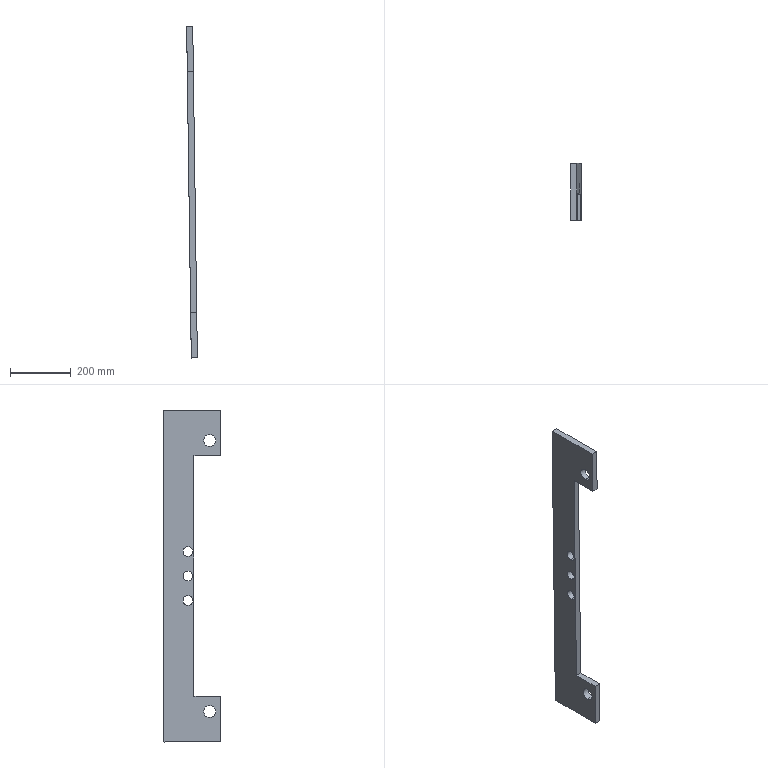Component | SolidWorks | DA-0220-Part3-1 | 1 solid | 22 faces | box 35.28 x 187.01 x 1090.17 mm | volume 2603445 mm3 | cylinder 12 | plane 10 | commonest cylinder face diameters 32 x6 40 x4 4 x2
build123d program:
from build123d import *

# Parameters (mm, degrees)
SKETCH1_W             = 1090
SKETCH1_H             = 100
BOSS_EXTRUDE1_DEPTH   = 20
FILLET1_R             = 2
SKETCH2_R             = 16
CUT_EXTRUDE2_DEPTH    = 548.654
SKETCH3_W             = 150
SKETCH3_H             = 87
BOSS_EXTRUDE1_2_DEPTH = 20
SKETCH4_R             = 20
CUT_EXTRUDE5_DEPTH    = 563.311


with BuildPart() as part:
    # Sketch1 → Boss-Extrude1 (new body)
    with BuildSketch(Plane.XY):
        Rectangle(SKETCH1_W, SKETCH1_H)
    extrude(amount=BOSS_EXTRUDE1_DEPTH)

    # Fillet1
    fillet1_edges = [part.edges().sort_by_distance(p)[0] for p in [
        (-545, 50, 10),
        (545, 50, 10),
    ]]
    fillet(fillet1_edges, radius=FILLET1_R)

    # Sketch2 → Cut-Extrude2 (cut, through all)
    with BuildSketch(Plane.XY.offset(20)):
        with Locations(Location((0, -30, 0), (0, 0, 180))):
            Circle(SKETCH2_R)
        with Locations((-80, -30)):
            Circle(SKETCH2_R)
        with Locations((80, -30)):
            Circle(SKETCH2_R)
    extrude(amount=-CUT_EXTRUDE2_DEPTH, mode=Mode.SUBTRACT)

    # Sketch3 → Boss-Extrude1_2 (add)
    with BuildSketch(Plane(origin=(0, 0, 0), x_dir=(-1, 0, 0), z_dir=(0, 0, -1))):
        with Locations((470, -93.5)):
            Rectangle(SKETCH3_W, SKETCH3_H)
        with Locations((-470, -93.5)):
            Rectangle(SKETCH3_W, SKETCH3_H)
    extrude(amount=-BOSS_EXTRUDE1_2_DEPTH)

    # Sketch4 → Cut-Extrude5 (cut, through all)
    with BuildSketch(Plane.XY.offset(20)):
        with Locations((-445, -102)):
            Circle(SKETCH4_R)
        with Locations((445, -102)):
            Circle(SKETCH4_R)
    extrude(amount=-CUT_EXTRUDE5_DEPTH, mode=Mode.SUBTRACT)


solid = part.part

# Placed as in the assembly
solid = solid.moved(Location((496.12, -63.852, 10.424), (178.341, -89.2, 178.341)))
STEP:
#1=CARTESIAN_POINT('',(18.98,-6.53,-16.331));
#2=VERTEX_POINT('',#1);
#3=CARTESIAN_POINT('',(19.002,-6.53,-17.906));
#4=VERTEX_POINT('',#3);
#5=CARTESIAN_POINT('',(18.991,-6.53,-17.119));
#6=DIRECTION('',(0.9999,0.000404,0.01395));
#7=DIRECTION('',(0.01395,0.00000282,-0.9999));
#8=AXIS2_PLACEMENT_3D('',#5,#6,#7);
#9=CIRCLE('',#8,0.7874);
#10=EDGE_CURVE('',#2,#4,#9,.T.);
#11=ORIENTED_EDGE('',*,*,#10,.F.);
#12=CARTESIAN_POINT('',(19.767,-6.53,-16.32));
#13=VERTEX_POINT('',#12);
#14=CARTESIAN_POINT('',(18.98,-6.53,-16.331));
#15=DIRECTION('',(0.9999,0.000404,0.01395));
#16=VECTOR('',#15,39.37);
#17=LINE('',#14,#16);
#18=EDGE_CURVE('',#2,#13,#17,.T.);
#19=ORIENTED_EDGE('',*,*,#18,.T.);
#20=CARTESIAN_POINT('',(19.789,-6.53,-17.895));
#21=VERTEX_POINT('',#20);
#22=CARTESIAN_POINT('',(19.778,-6.53,-17.108));
#23=DIRECTION('',(0.9999,0.000404,0.01395));
#24=DIRECTION('',(0.01395,0.00000282,-0.9999));
#25=AXIS2_PLACEMENT_3D('',#22,#23,#24);
#26=CIRCLE('',#25,0.7874);
#27=EDGE_CURVE('',#13,#21,#26,.T.);
#28=ORIENTED_EDGE('',*,*,#27,.T.);
#29=CARTESIAN_POINT('',(19.002,-6.53,-17.906));
#30=DIRECTION('',(0.9999,0.000404,0.01395));
#31=VECTOR('',#30,39.37);
#32=LINE('',#29,#31);
#33=EDGE_CURVE('',#4,#21,#32,.T.);
#34=ORIENTED_EDGE('',*,*,#33,.F.);
#35=EDGE_LOOP('',(#11,#19,#28,#34));
#36=FACE_OUTER_BOUND('',#35,.T.);
#37=CARTESIAN_POINT('',(18.991,-6.53,-17.119));
#38=DIRECTION('',(0.9999,0.000404,0.01395));
#39=DIRECTION('',(0.01395,0.00000282,-0.9999));
#40=AXIS2_PLACEMENT_3D('',#37,#38,#39);
#41=CYLINDRICAL_SURFACE('',#40,0.7874);
#42=ADVANCED_FACE('',(#36),#41,.F.);
#43=CARTESIAN_POINT('',(18.491,-6.53,18.705));
#44=VERTEX_POINT('',#43);
#45=CARTESIAN_POINT('',(18.513,-6.53,17.13));
#46=VERTEX_POINT('',#45);
#47=CARTESIAN_POINT('',(18.502,-6.53,17.917));
#48=DIRECTION('',(0.9999,0.000404,0.01395));
#49=DIRECTION('',(0.01395,0.00000282,-0.9999));
#50=AXIS2_PLACEMENT_3D('',#47,#48,#49);
#51=CIRCLE('',#50,0.7874);
#52=EDGE_CURVE('',#44,#46,#51,.T.);
#53=ORIENTED_EDGE('',*,*,#52,.F.);
#54=CARTESIAN_POINT('',(19.278,-6.53,18.716));
#55=VERTEX_POINT('',#54);
#56=CARTESIAN_POINT('',(18.491,-6.53,18.705));
#57=DIRECTION('',(0.9999,0.000404,0.01395));
#58=VECTOR('',#57,39.37);
#59=LINE('',#56,#58);
#60=EDGE_CURVE('',#44,#55,#59,.T.);
#61=ORIENTED_EDGE('',*,*,#60,.T.);
#62=CARTESIAN_POINT('',(19.3,-6.53,17.141));
#63=VERTEX_POINT('',#62);
#64=CARTESIAN_POINT('',(19.289,-6.53,17.928));
#65=DIRECTION('',(0.9999,0.000404,0.01395));
#66=DIRECTION('',(0.01395,0.00000282,-0.9999));
#67=AXIS2_PLACEMENT_3D('',#64,#65,#66);
#68=CIRCLE('',#67,0.7874);
#69=EDGE_CURVE('',#55,#63,#68,.T.);
#70=ORIENTED_EDGE('',*,*,#69,.T.);
#71=CARTESIAN_POINT('',(18.513,-6.53,17.13));
#72=DIRECTION('',(0.9999,0.000404,0.01395));
#73=VECTOR('',#72,39.37);
#74=LINE('',#71,#73);
#75=EDGE_CURVE('',#46,#63,#74,.T.);
#76=ORIENTED_EDGE('',*,*,#75,.F.);
#77=EDGE_LOOP('',(#53,#61,#70,#76));
#78=FACE_OUTER_BOUND('',#77,.T.);
#79=CARTESIAN_POINT('',(18.502,-6.53,17.917));
#80=DIRECTION('',(0.9999,0.000404,0.01395));
#81=DIRECTION('',(0.01395,0.00000282,-0.9999));
#82=AXIS2_PLACEMENT_3D('',#79,#80,#81);
#83=CYLINDRICAL_SURFACE('',#82,0.7874);
#84=ADVANCED_FACE('',(#78),#83,.F.);
#85=CARTESIAN_POINT('',(18.781,-3.695,-2.12));
#86=VERTEX_POINT('',#85);
#87=CARTESIAN_POINT('',(18.798,-3.695,-3.38));
#88=VERTEX_POINT('',#87);
#89=CARTESIAN_POINT('',(18.789,-3.695,-2.75));
#90=DIRECTION('',(0.9999,0.000404,0.01395));
#91=DIRECTION('',(0.01395,0.00000282,-0.9999));
#92=AXIS2_PLACEMENT_3D('',#89,#90,#91);
#93=CIRCLE('',#92,0.6299);
#94=EDGE_CURVE('',#86,#88,#93,.T.);
#95=ORIENTED_EDGE('',*,*,#94,.F.);
#96=CARTESIAN_POINT('',(19.568,-3.695,-2.109));
#97=VERTEX_POINT('',#96);
#98=CARTESIAN_POINT('',(18.781,-3.695,-2.12));
#99=DIRECTION('',(0.9999,0.000404,0.01395));
#100=VECTOR('',#99,39.37);
#101=LINE('',#98,#100);
#102=EDGE_CURVE('',#86,#97,#101,.T.);
#103=ORIENTED_EDGE('',*,*,#102,.T.);
#104=CARTESIAN_POINT('',(19.585,-3.695,-3.369));
#105=VERTEX_POINT('',#104);
#106=CARTESIAN_POINT('',(19.577,-3.695,-2.739));
#107=DIRECTION('',(0.9999,0.000404,0.01395));
#108=DIRECTION('',(0.01395,0.00000282,-0.9999));
#109=AXIS2_PLACEMENT_3D('',#106,#107,#108);
#110=CIRCLE('',#109,0.6299);
#111=EDGE_CURVE('',#97,#105,#110,.T.);
#112=ORIENTED_EDGE('',*,*,#111,.T.);
#113=CARTESIAN_POINT('',(18.798,-3.695,-3.38));
#114=DIRECTION('',(0.9999,0.000404,0.01395));
#115=VECTOR('',#114,39.37);
#116=LINE('',#113,#115);
#117=EDGE_CURVE('',#88,#105,#116,.T.);
#118=ORIENTED_EDGE('',*,*,#117,.F.);
#119=EDGE_LOOP('',(#95,#103,#112,#118));
#120=FACE_OUTER_BOUND('',#119,.T.);
#121=CARTESIAN_POINT('',(18.789,-3.695,-2.75));
#122=DIRECTION('',(0.9999,0.000404,0.01395));
#123=DIRECTION('',(0.01395,0.00000282,-0.9999));
#124=AXIS2_PLACEMENT_3D('',#121,#122,#123);
#125=CYLINDRICAL_SURFACE('',#124,0.6299);
#126=ADVANCED_FACE('',(#120),#125,.F.);
#127=CARTESIAN_POINT('',(18.693,-3.695,4.179));
#128=VERTEX_POINT('',#127);
#129=CARTESIAN_POINT('',(18.71,-3.695,2.919));
#130=VERTEX_POINT('',#129);
#131=CARTESIAN_POINT('',(18.701,-3.695,3.549));
#132=DIRECTION('',(0.9999,0.000404,0.01395));
#133=DIRECTION('',(0.01395,0.00000282,-0.9999));
#134=AXIS2_PLACEMENT_3D('',#131,#132,#133);
#135=CIRCLE('',#134,0.6299);
#136=EDGE_CURVE('',#128,#130,#135,.T.);
#137=ORIENTED_EDGE('',*,*,#136,.F.);
#138=CARTESIAN_POINT('',(19.48,-3.695,4.19));
#139=VERTEX_POINT('',#138);
#140=CARTESIAN_POINT('',(18.693,-3.695,4.179));
#141=DIRECTION('',(0.9999,0.000404,0.01395));
#142=VECTOR('',#141,39.37);
#143=LINE('',#140,#142);
#144=EDGE_CURVE('',#128,#139,#143,.T.);
#145=ORIENTED_EDGE('',*,*,#144,.T.);
#146=CARTESIAN_POINT('',(19.498,-3.695,2.93));
#147=VERTEX_POINT('',#146);
#148=CARTESIAN_POINT('',(19.489,-3.695,3.56));
#149=DIRECTION('',(0.9999,0.000404,0.01395));
#150=DIRECTION('',(0.01395,0.00000282,-0.9999));
#151=AXIS2_PLACEMENT_3D('',#148,#149,#150);
#152=CIRCLE('',#151,0.6299);
#153=EDGE_CURVE('',#139,#147,#152,.T.);
#154=ORIENTED_EDGE('',*,*,#153,.T.);
#155=CARTESIAN_POINT('',(18.71,-3.695,2.919));
#156=DIRECTION('',(0.9999,0.000404,0.01395));
#157=VECTOR('',#156,39.37);
#158=LINE('',#155,#157);
#159=EDGE_CURVE('',#130,#147,#158,.T.);
#160=ORIENTED_EDGE('',*,*,#159,.F.);
#161=EDGE_LOOP('',(#137,#145,#154,#160));
#162=FACE_OUTER_BOUND('',#161,.T.);
#163=CARTESIAN_POINT('',(18.701,-3.695,3.549));
#164=DIRECTION('',(0.9999,0.000404,0.01395));
#165=DIRECTION('',(0.01395,0.00000282,-0.9999));
#166=AXIS2_PLACEMENT_3D('',#163,#164,#165);
#167=CYLINDRICAL_SURFACE('',#166,0.6299);
#168=ADVANCED_FACE('',(#162),#167,.F.);
#169=CARTESIAN_POINT('',(18.737,-3.695,1.029));
#170=VERTEX_POINT('',#169);
#171=CARTESIAN_POINT('',(18.754,-3.695,-0.2304));
#172=VERTEX_POINT('',#171);
#173=CARTESIAN_POINT('',(18.745,-3.695,0.3994));
#174=DIRECTION('',(0.9999,0.000404,0.01395));
#175=DIRECTION('',(-0.01395,-0.00000282,0.9999));
#176=AXIS2_PLACEMENT_3D('',#173,#174,#175);
#177=CIRCLE('',#176,0.6299);
#178=EDGE_CURVE('',#170,#172,#177,.T.);
#179=ORIENTED_EDGE('',*,*,#178,.F.);
#180=CARTESIAN_POINT('',(19.524,-3.695,1.04));
#181=VERTEX_POINT('',#180);
#182=CARTESIAN_POINT('',(18.737,-3.695,1.029));
#183=DIRECTION('',(0.9999,0.000404,0.01395));
#184=VECTOR('',#183,39.37);
#185=LINE('',#182,#184);
#186=EDGE_CURVE('',#170,#181,#185,.T.);
#187=ORIENTED_EDGE('',*,*,#186,.T.);
#188=CARTESIAN_POINT('',(19.542,-3.695,-0.2194));
#189=VERTEX_POINT('',#188);
#190=CARTESIAN_POINT('',(19.533,-3.695,0.4104));
#191=DIRECTION('',(0.9999,0.000404,0.01395));
#192=DIRECTION('',(-0.01395,-0.00000282,0.9999));
#193=AXIS2_PLACEMENT_3D('',#190,#191,#192);
#194=CIRCLE('',#193,0.6299);
#195=EDGE_CURVE('',#181,#189,#194,.T.);
#196=ORIENTED_EDGE('',*,*,#195,.T.);
#197=CARTESIAN_POINT('',(18.754,-3.695,-0.2304));
#198=DIRECTION('',(0.9999,0.000404,0.01395));
#199=VECTOR('',#198,39.37);
#200=LINE('',#197,#199);
#201=EDGE_CURVE('',#172,#189,#200,.T.);
#202=ORIENTED_EDGE('',*,*,#201,.F.);
#203=EDGE_LOOP('',(#179,#187,#196,#202));
#204=FACE_OUTER_BOUND('',#203,.T.);
#205=CARTESIAN_POINT('',(18.745,-3.695,0.3994));
#206=DIRECTION('',(0.9999,0.000404,0.01395));
#207=DIRECTION('',(0.01395,0.00000282,-0.9999));
#208=AXIS2_PLACEMENT_3D('',#205,#206,#207);
#209=CYLINDRICAL_SURFACE('',#208,0.6299);
#210=ADVANCED_FACE('',(#204),#209,.F.);
#211=CARTESIAN_POINT('',(19.047,-7.908,-21.055));
#212=VERTEX_POINT('',#211);
#213=CARTESIAN_POINT('',(19.044,-0.6243,-21.055));
#214=VERTEX_POINT('',#213);
#215=CARTESIAN_POINT('',(19.044,-0.5456,-21.055));
#216=DIRECTION('',(-0.000404,1.,-0.00000282));
#217=VECTOR('',#216,39.37);
#218=LINE('',#215,#217);
#219=EDGE_CURVE('',#212,#214,#218,.T.);
#220=ORIENTED_EDGE('',*,*,#219,.T.);
#221=CARTESIAN_POINT('',(19.831,-0.624,-21.044));
#222=VERTEX_POINT('',#221);
#223=CARTESIAN_POINT('',(19.831,-0.624,-21.044));
#224=DIRECTION('',(0.9999,0.000404,0.01395));
#225=VECTOR('',#224,39.37);
#226=LINE('',#223,#225);
#227=EDGE_CURVE('',#214,#222,#226,.T.);
#228=ORIENTED_EDGE('',*,*,#227,.T.);
#229=CARTESIAN_POINT('',(19.834,-7.907,-21.044));
#230=VERTEX_POINT('',#229);
#231=CARTESIAN_POINT('',(19.831,-0.5453,-21.044));
#232=DIRECTION('',(-0.000404,1.,-0.00000282));
#233=VECTOR('',#232,39.37);
#234=LINE('',#231,#233);
#235=EDGE_CURVE('',#230,#222,#234,.T.);
#236=ORIENTED_EDGE('',*,*,#235,.F.);
#237=CARTESIAN_POINT('',(26.66,-7.905,-20.949));
#238=DIRECTION('',(-0.9999,-0.000404,-0.01395));
#239=VECTOR('',#238,39.37);
#240=LINE('',#237,#239);
#241=EDGE_CURVE('',#230,#212,#240,.T.);
#242=ORIENTED_EDGE('',*,*,#241,.T.);
#243=EDGE_LOOP('',(#220,#228,#236,#242));
#244=FACE_OUTER_BOUND('',#243,.T.);
#245=CARTESIAN_POINT('',(19.831,-0.5453,-21.044));
#246=DIRECTION('',(-0.01395,-0.00000282,0.9999));
#247=DIRECTION('',(0.9999,0.000404,0.01395));
#248=AXIS2_PLACEMENT_3D('',#245,#246,#247);
#249=PLANE('',#248);
#250=ADVANCED_FACE('',(#244),#249,.F.);
#251=CARTESIAN_POINT('',(19.042,-0.5456,-20.976));
#252=VERTEX_POINT('',#251);
#253=CARTESIAN_POINT('',(18.446,-0.5457,21.775));
#254=VERTEX_POINT('',#253);
#255=CARTESIAN_POINT('',(18.445,-0.5457,21.854));
#256=DIRECTION('',(-0.01395,-0.00000282,0.9999));
#257=VECTOR('',#256,39.37);
#258=LINE('',#255,#257);
#259=EDGE_CURVE('',#252,#254,#258,.T.);
#260=ORIENTED_EDGE('',*,*,#259,.T.);
#261=CARTESIAN_POINT('',(19.233,-0.5454,21.786));
#262=VERTEX_POINT('',#261);
#263=CARTESIAN_POINT('',(19.233,-0.5454,21.786));
#264=DIRECTION('',(0.9999,0.000404,0.01395));
#265=VECTOR('',#264,39.37);
#266=LINE('',#263,#265);
#267=EDGE_CURVE('',#254,#262,#266,.T.);
#268=ORIENTED_EDGE('',*,*,#267,.T.);
#269=CARTESIAN_POINT('',(19.83,-0.5453,-20.965));
#270=VERTEX_POINT('',#269);
#271=CARTESIAN_POINT('',(19.232,-0.5454,21.865));
#272=DIRECTION('',(-0.01395,-0.00000282,0.9999));
#273=VECTOR('',#272,39.37);
#274=LINE('',#271,#273);
#275=EDGE_CURVE('',#270,#262,#274,.T.);
#276=ORIENTED_EDGE('',*,*,#275,.F.);
#277=CARTESIAN_POINT('',(19.83,-0.5453,-20.965));
#278=DIRECTION('',(-0.9999,-0.000404,-0.01395));
#279=VECTOR('',#278,39.37);
#280=LINE('',#277,#279);
#281=EDGE_CURVE('',#270,#252,#280,.T.);
#282=ORIENTED_EDGE('',*,*,#281,.T.);
#283=EDGE_LOOP('',(#260,#268,#276,#282));
#284=FACE_OUTER_BOUND('',#283,.T.);
#285=CARTESIAN_POINT('',(19.232,-0.5454,21.865));
#286=DIRECTION('',(0.000404,-1.,0.00000282));
#287=DIRECTION('',(-0.9999,-0.000404,-0.01395));
#288=AXIS2_PLACEMENT_3D('',#285,#286,#287);
#289=PLANE('',#288);
#290=ADVANCED_FACE('',(#284),#289,.F.);
#291=CARTESIAN_POINT('',(19.232,-0.6242,21.865));
#292=VERTEX_POINT('',#291);
#293=CARTESIAN_POINT('',(19.235,-7.908,21.865));
#294=VERTEX_POINT('',#293);
#295=CARTESIAN_POINT('',(19.232,-0.5454,21.865));
#296=DIRECTION('',(0.000404,-1.,0.00000282));
#297=VECTOR('',#296,39.37);
#298=LINE('',#295,#297);
#299=EDGE_CURVE('',#292,#294,#298,.T.);
#300=ORIENTED_EDGE('',*,*,#299,.F.);
#301=CARTESIAN_POINT('',(18.445,-0.6245,21.854));
#302=VERTEX_POINT('',#301);
#303=CARTESIAN_POINT('',(19.232,-0.6242,21.865));
#304=DIRECTION('',(-0.9999,-0.000404,-0.01395));
#305=VECTOR('',#304,39.37);
#306=LINE('',#303,#305);
#307=EDGE_CURVE('',#292,#302,#306,.T.);
#308=ORIENTED_EDGE('',*,*,#307,.T.);
#309=CARTESIAN_POINT('',(18.448,-7.908,21.854));
#310=VERTEX_POINT('',#309);
#311=CARTESIAN_POINT('',(18.445,-0.5457,21.854));
#312=DIRECTION('',(0.000404,-1.,0.00000282));
#313=VECTOR('',#312,39.37);
#314=LINE('',#311,#313);
#315=EDGE_CURVE('',#302,#310,#314,.T.);
#316=ORIENTED_EDGE('',*,*,#315,.T.);
#317=CARTESIAN_POINT('',(26.061,-7.905,21.96));
#318=DIRECTION('',(-0.9999,-0.000404,-0.01395));
#319=VECTOR('',#318,39.37);
#320=LINE('',#317,#319);
#321=EDGE_CURVE('',#294,#310,#320,.T.);
#322=ORIENTED_EDGE('',*,*,#321,.F.);
#323=EDGE_LOOP('',(#300,#308,#316,#322));
#324=FACE_OUTER_BOUND('',#323,.T.);
#325=CARTESIAN_POINT('',(19.232,-0.5454,21.865));
#326=DIRECTION('',(0.01395,0.00000282,-0.9999));
#327=DIRECTION('',(-0.9999,-0.000404,-0.01395));
#328=AXIS2_PLACEMENT_3D('',#325,#326,#327);
#329=PLANE('',#328);
#330=ADVANCED_FACE('',(#324),#329,.F.);
#331=CARTESIAN_POINT('',(18.529,-4.483,15.949));
#332=VERTEX_POINT('',#331);
#333=CARTESIAN_POINT('',(18.963,-4.483,-15.15));
#334=VERTEX_POINT('',#333);
#335=CARTESIAN_POINT('',(18.446,-4.483,21.854));
#336=DIRECTION('',(0.01395,0.00000282,-0.9999));
#337=VECTOR('',#336,39.37);
#338=LINE('',#335,#337);
#339=EDGE_CURVE('',#332,#334,#338,.T.);
#340=ORIENTED_EDGE('',*,*,#339,.T.);
#341=CARTESIAN_POINT('',(19.75,-4.482,-15.139));
#342=VERTEX_POINT('',#341);
#343=CARTESIAN_POINT('',(26.576,-4.48,-15.044));
#344=DIRECTION('',(-0.9999,-0.000404,-0.01395));
#345=VECTOR('',#344,39.37);
#346=LINE('',#343,#345);
#347=EDGE_CURVE('',#342,#334,#346,.T.);
#348=ORIENTED_EDGE('',*,*,#347,.F.);
#349=CARTESIAN_POINT('',(19.316,-4.482,15.96));
#350=VERTEX_POINT('',#349);
#351=CARTESIAN_POINT('',(19.234,-4.482,21.865));
#352=DIRECTION('',(0.01395,0.00000282,-0.9999));
#353=VECTOR('',#352,39.37);
#354=LINE('',#351,#353);
#355=EDGE_CURVE('',#350,#342,#354,.T.);
#356=ORIENTED_EDGE('',*,*,#355,.F.);
#357=CARTESIAN_POINT('',(26.142,-4.48,16.055));
#358=DIRECTION('',(-0.9999,-0.000404,-0.01395));
#359=VECTOR('',#358,39.37);
#360=LINE('',#357,#359);
#361=EDGE_CURVE('',#350,#332,#360,.T.);
#362=ORIENTED_EDGE('',*,*,#361,.T.);
#363=EDGE_LOOP('',(#340,#348,#356,#362));
#364=FACE_OUTER_BOUND('',#363,.T.);
#365=CARTESIAN_POINT('',(19.234,-4.482,21.865));
#366=DIRECTION('',(-0.000404,1.,-0.00000282));
#367=DIRECTION('',(0.9999,0.000404,0.01395));
#368=AXIS2_PLACEMENT_3D('',#365,#366,#367);
#369=PLANE('',#368);
#370=ADVANCED_FACE('',(#364),#369,.F.);
#371=CARTESIAN_POINT('',(19.778,-6.53,-17.108));
#372=DIRECTION('',(0.9999,0.000404,0.01395));
#373=DIRECTION('',(0.01395,0.00000282,-0.9999));
#374=AXIS2_PLACEMENT_3D('',#371,#372,#373);
#375=CIRCLE('',#374,0.7874);
#376=EDGE_CURVE('',#21,#13,#375,.T.);
#377=ORIENTED_EDGE('',*,*,#376,.F.);
#378=ORIENTED_EDGE('',*,*,#27,.F.);
#379=EDGE_LOOP('',(#377,#378));
#380=FACE_BOUND('',#379,.T.);
#381=CARTESIAN_POINT('',(19.289,-6.53,17.928));
#382=DIRECTION('',(0.9999,0.000404,0.01395));
#383=DIRECTION('',(0.01395,0.00000282,-0.9999));
#384=AXIS2_PLACEMENT_3D('',#381,#382,#383);
#385=CIRCLE('',#384,0.7874);
#386=EDGE_CURVE('',#63,#55,#385,.T.);
#387=ORIENTED_EDGE('',*,*,#386,.F.);
#388=ORIENTED_EDGE('',*,*,#69,.F.);
#389=EDGE_LOOP('',(#387,#388));
#390=FACE_BOUND('',#389,.T.);
#391=CARTESIAN_POINT('',(19.577,-3.695,-2.739));
#392=DIRECTION('',(0.9999,0.000404,0.01395));
#393=DIRECTION('',(0.01395,0.00000282,-0.9999));
#394=AXIS2_PLACEMENT_3D('',#391,#392,#393);
#395=CIRCLE('',#394,0.6299);
#396=EDGE_CURVE('',#105,#97,#395,.T.);
#397=ORIENTED_EDGE('',*,*,#396,.F.);
#398=ORIENTED_EDGE('',*,*,#111,.F.);
#399=EDGE_LOOP('',(#397,#398));
#400=FACE_BOUND('',#399,.T.);
#401=CARTESIAN_POINT('',(19.489,-3.695,3.56));
#402=DIRECTION('',(0.9999,0.000404,0.01395));
#403=DIRECTION('',(0.01395,0.00000282,-0.9999));
#404=AXIS2_PLACEMENT_3D('',#401,#402,#403);
#405=CIRCLE('',#404,0.6299);
#406=EDGE_CURVE('',#147,#139,#405,.T.);
#407=ORIENTED_EDGE('',*,*,#406,.F.);
#408=ORIENTED_EDGE('',*,*,#153,.F.);
#409=EDGE_LOOP('',(#407,#408));
#410=FACE_BOUND('',#409,.T.);
#411=CARTESIAN_POINT('',(19.533,-3.695,0.4104));
#412=DIRECTION('',(0.9999,0.000404,0.01395));
#413=DIRECTION('',(-0.01395,-0.00000282,0.9999));
#414=AXIS2_PLACEMENT_3D('',#411,#412,#413);
#415=CIRCLE('',#414,0.6299);
#416=EDGE_CURVE('',#189,#181,#415,.T.);
#417=ORIENTED_EDGE('',*,*,#416,.F.);
#418=ORIENTED_EDGE('',*,*,#195,.F.);
#419=EDGE_LOOP('',(#417,#418));
#420=FACE_BOUND('',#419,.T.);
#421=ORIENTED_EDGE('',*,*,#275,.T.);
#422=CARTESIAN_POINT('',(19.233,-0.6242,21.786));
#423=DIRECTION('',(0.9999,0.000404,0.01395));
#424=DIRECTION('',(0.01395,0.00000282,-0.9999));
#425=AXIS2_PLACEMENT_3D('',#422,#423,#424);
#426=CIRCLE('',#425,0.07874);
#427=EDGE_CURVE('',#262,#292,#426,.T.);
#428=ORIENTED_EDGE('',*,*,#427,.T.);
#429=ORIENTED_EDGE('',*,*,#299,.T.);
#430=CARTESIAN_POINT('',(19.317,-7.908,15.96));
#431=VERTEX_POINT('',#430);
#432=CARTESIAN_POINT('',(19.317,-7.908,15.96));
#433=DIRECTION('',(-0.01395,-0.00000282,0.9999));
#434=VECTOR('',#433,39.37);
#435=LINE('',#432,#434);
#436=EDGE_CURVE('',#431,#294,#435,.T.);
#437=ORIENTED_EDGE('',*,*,#436,.F.);
#438=CARTESIAN_POINT('',(19.317,-7.908,15.96));
#439=DIRECTION('',(0.000404,-1.,0.00000282));
#440=VECTOR('',#439,39.37);
#441=LINE('',#438,#440);
#442=EDGE_CURVE('',#350,#431,#441,.T.);
#443=ORIENTED_EDGE('',*,*,#442,.F.);
#444=ORIENTED_EDGE('',*,*,#355,.T.);
#445=CARTESIAN_POINT('',(19.751,-7.908,-15.139));
#446=VERTEX_POINT('',#445);
#447=CARTESIAN_POINT('',(19.751,-7.908,-15.139));
#448=DIRECTION('',(-0.000404,1.,-0.00000282));
#449=VECTOR('',#448,39.37);
#450=LINE('',#447,#449);
#451=EDGE_CURVE('',#446,#342,#450,.T.);
#452=ORIENTED_EDGE('',*,*,#451,.F.);
#453=CARTESIAN_POINT('',(19.751,-7.908,-15.139));
#454=DIRECTION('',(-0.01395,-0.00000282,0.9999));
#455=VECTOR('',#454,39.37);
#456=LINE('',#453,#455);
#457=EDGE_CURVE('',#230,#446,#456,.T.);
#458=ORIENTED_EDGE('',*,*,#457,.F.);
#459=ORIENTED_EDGE('',*,*,#235,.T.);
#460=CARTESIAN_POINT('',(19.83,-0.624,-20.965));
#461=DIRECTION('',(0.9999,0.000404,0.01395));
#462=DIRECTION('',(0.01395,0.00000282,-0.9999));
#463=AXIS2_PLACEMENT_3D('',#460,#461,#462);
#464=CIRCLE('',#463,0.07874);
#465=EDGE_CURVE('',#222,#270,#464,.T.);
#466=ORIENTED_EDGE('',*,*,#465,.T.);
#467=EDGE_LOOP('',(#421,#428,#429,#437,#443,#444,#452,#458,#459,#466));
#468=FACE_OUTER_BOUND('',#467,.T.);
#469=CARTESIAN_POINT('',(19.832,-4.482,-21.044));
#470=DIRECTION('',(0.9999,0.000404,0.01395));
#471=DIRECTION('',(0.01395,0.00000282,-0.9999));
#472=AXIS2_PLACEMENT_3D('',#469,#470,#471);
#473=PLANE('',#472);
#474=ADVANCED_FACE('',(#380,#390,#400,#410,#420,#468),#473,.T.);
#475=CARTESIAN_POINT('',(18.991,-6.53,-17.119));
#476=DIRECTION('',(0.9999,0.000404,0.01395));
#477=DIRECTION('',(0.01395,0.00000282,-0.9999));
#478=AXIS2_PLACEMENT_3D('',#475,#476,#477);
#479=CIRCLE('',#478,0.7874);
#480=EDGE_CURVE('',#4,#2,#479,.T.);
#481=ORIENTED_EDGE('',*,*,#480,.T.);
#482=ORIENTED_EDGE('',*,*,#10,.T.);
#483=EDGE_LOOP('',(#481,#482));
#484=FACE_BOUND('',#483,.T.);
#485=CARTESIAN_POINT('',(18.502,-6.53,17.917));
#486=DIRECTION('',(0.9999,0.000404,0.01395));
#487=DIRECTION('',(0.01395,0.00000282,-0.9999));
#488=AXIS2_PLACEMENT_3D('',#485,#486,#487);
#489=CIRCLE('',#488,0.7874);
#490=EDGE_CURVE('',#46,#44,#489,.T.);
#491=ORIENTED_EDGE('',*,*,#490,.T.);
#492=ORIENTED_EDGE('',*,*,#52,.T.);
#493=EDGE_LOOP('',(#491,#492));
#494=FACE_BOUND('',#493,.T.);
#495=CARTESIAN_POINT('',(18.789,-3.695,-2.75));
#496=DIRECTION('',(0.9999,0.000404,0.01395));
#497=DIRECTION('',(0.01395,0.00000282,-0.9999));
#498=AXIS2_PLACEMENT_3D('',#495,#496,#497);
#499=CIRCLE('',#498,0.6299);
#500=EDGE_CURVE('',#88,#86,#499,.T.);
#501=ORIENTED_EDGE('',*,*,#500,.T.);
#502=ORIENTED_EDGE('',*,*,#94,.T.);
#503=EDGE_LOOP('',(#501,#502));
#504=FACE_BOUND('',#503,.T.);
#505=CARTESIAN_POINT('',(18.701,-3.695,3.549));
#506=DIRECTION('',(0.9999,0.000404,0.01395));
#507=DIRECTION('',(0.01395,0.00000282,-0.9999));
#508=AXIS2_PLACEMENT_3D('',#505,#506,#507);
#509=CIRCLE('',#508,0.6299);
#510=EDGE_CURVE('',#130,#128,#509,.T.);
#511=ORIENTED_EDGE('',*,*,#510,.T.);
#512=ORIENTED_EDGE('',*,*,#136,.T.);
#513=EDGE_LOOP('',(#511,#512));
#514=FACE_BOUND('',#513,.T.);
#515=CARTESIAN_POINT('',(18.745,-3.695,0.3994));
#516=DIRECTION('',(0.9999,0.000404,0.01395));
#517=DIRECTION('',(-0.01395,-0.00000282,0.9999));
#518=AXIS2_PLACEMENT_3D('',#515,#516,#517);
#519=CIRCLE('',#518,0.6299);
#520=EDGE_CURVE('',#172,#170,#519,.T.);
#521=ORIENTED_EDGE('',*,*,#520,.T.);
#522=ORIENTED_EDGE('',*,*,#178,.T.);
#523=EDGE_LOOP('',(#521,#522));
#524=FACE_BOUND('',#523,.T.);
#525=ORIENTED_EDGE('',*,*,#315,.F.);
#526=CARTESIAN_POINT('',(18.446,-0.6245,21.775));
#527=DIRECTION('',(-0.9999,-0.000404,-0.01395));
#528=DIRECTION('',(0.01395,0.00000282,-0.9999));
#529=AXIS2_PLACEMENT_3D('',#526,#527,#528);
#530=CIRCLE('',#529,0.07874);
#531=EDGE_CURVE('',#302,#254,#530,.T.);
#532=ORIENTED_EDGE('',*,*,#531,.T.);
#533=ORIENTED_EDGE('',*,*,#259,.F.);
#534=CARTESIAN_POINT('',(19.042,-0.6243,-20.976));
#535=DIRECTION('',(-0.9999,-0.000404,-0.01395));
#536=DIRECTION('',(0.01395,0.00000282,-0.9999));
#537=AXIS2_PLACEMENT_3D('',#534,#535,#536);
#538=CIRCLE('',#537,0.07874);
#539=EDGE_CURVE('',#252,#214,#538,.T.);
#540=ORIENTED_EDGE('',*,*,#539,.T.);
#541=ORIENTED_EDGE('',*,*,#219,.F.);
#542=CARTESIAN_POINT('',(18.964,-7.908,-15.15));
#543=VERTEX_POINT('',#542);
#544=CARTESIAN_POINT('',(18.964,-7.908,-15.15));
#545=DIRECTION('',(-0.01395,-0.00000282,0.9999));
#546=VECTOR('',#545,39.37);
#547=LINE('',#544,#546);
#548=EDGE_CURVE('',#212,#543,#547,.T.);
#549=ORIENTED_EDGE('',*,*,#548,.T.);
#550=CARTESIAN_POINT('',(18.964,-7.908,-15.15));
#551=DIRECTION('',(-0.000404,1.,-0.00000282));
#552=VECTOR('',#551,39.37);
#553=LINE('',#550,#552);
#554=EDGE_CURVE('',#543,#334,#553,.T.);
#555=ORIENTED_EDGE('',*,*,#554,.T.);
#556=ORIENTED_EDGE('',*,*,#339,.F.);
#557=CARTESIAN_POINT('',(18.53,-7.908,15.949));
#558=VERTEX_POINT('',#557);
#559=CARTESIAN_POINT('',(18.53,-7.908,15.949));
#560=DIRECTION('',(0.000404,-1.,0.00000282));
#561=VECTOR('',#560,39.37);
#562=LINE('',#559,#561);
#563=EDGE_CURVE('',#332,#558,#562,.T.);
#564=ORIENTED_EDGE('',*,*,#563,.T.);
#565=CARTESIAN_POINT('',(18.53,-7.908,15.949));
#566=DIRECTION('',(-0.01395,-0.00000282,0.9999));
#567=VECTOR('',#566,39.37);
#568=LINE('',#565,#567);
#569=EDGE_CURVE('',#558,#310,#568,.T.);
#570=ORIENTED_EDGE('',*,*,#569,.T.);
#571=EDGE_LOOP('',(#525,#532,#533,#540,#541,#549,#555,#556,#564,#570));
#572=FACE_OUTER_BOUND('',#571,.T.);
#573=CARTESIAN_POINT('',(19.045,-4.483,-21.055));
#574=DIRECTION('',(0.9999,0.000404,0.01395));
#575=DIRECTION('',(0.01395,0.00000282,-0.9999));
#576=AXIS2_PLACEMENT_3D('',#573,#574,#575);
#577=PLANE('',#576);
#578=ADVANCED_FACE('',(#484,#494,#504,#514,#524,#572),#577,.F.);
#579=ORIENTED_EDGE('',*,*,#427,.F.);
#580=ORIENTED_EDGE('',*,*,#267,.F.);
#581=ORIENTED_EDGE('',*,*,#531,.F.);
#582=ORIENTED_EDGE('',*,*,#307,.F.);
#583=EDGE_LOOP('',(#579,#580,#581,#582));
#584=FACE_OUTER_BOUND('',#583,.T.);
#585=CARTESIAN_POINT('',(19.233,-0.6242,21.786));
#586=DIRECTION('',(-0.9999,-0.000404,-0.01395));
#587=DIRECTION('',(-0.01395,-0.00000282,0.9999));
#588=AXIS2_PLACEMENT_3D('',#585,#586,#587);
#589=CYLINDRICAL_SURFACE('',#588,0.07874);
#590=ADVANCED_FACE('',(#584),#589,.T.);
#591=ORIENTED_EDGE('',*,*,#465,.F.);
#592=ORIENTED_EDGE('',*,*,#227,.F.);
#593=ORIENTED_EDGE('',*,*,#539,.F.);
#594=ORIENTED_EDGE('',*,*,#281,.F.);
#595=EDGE_LOOP('',(#591,#592,#593,#594));
#596=FACE_OUTER_BOUND('',#595,.T.);
#597=CARTESIAN_POINT('',(19.83,-0.624,-20.965));
#598=DIRECTION('',(-0.9999,-0.000404,-0.01395));
#599=DIRECTION('',(-0.01395,-0.00000282,0.9999));
#600=AXIS2_PLACEMENT_3D('',#597,#598,#599);
#601=CYLINDRICAL_SURFACE('',#600,0.07874);
#602=ADVANCED_FACE('',(#596),#601,.T.);
#603=ORIENTED_EDGE('',*,*,#186,.F.);
#604=ORIENTED_EDGE('',*,*,#520,.F.);
#605=ORIENTED_EDGE('',*,*,#201,.T.);
#606=ORIENTED_EDGE('',*,*,#416,.T.);
#607=EDGE_LOOP('',(#603,#604,#605,#606));
#608=FACE_OUTER_BOUND('',#607,.T.);
#609=CARTESIAN_POINT('',(18.745,-3.695,0.3994));
#610=DIRECTION('',(0.9999,0.000404,0.01395));
#611=DIRECTION('',(0.01395,0.00000282,-0.9999));
#612=AXIS2_PLACEMENT_3D('',#609,#610,#611);
#613=CYLINDRICAL_SURFACE('',#612,0.6299);
#614=ADVANCED_FACE('',(#608),#613,.F.);
#615=ORIENTED_EDGE('',*,*,#144,.F.);
#616=ORIENTED_EDGE('',*,*,#510,.F.);
#617=ORIENTED_EDGE('',*,*,#159,.T.);
#618=ORIENTED_EDGE('',*,*,#406,.T.);
#619=EDGE_LOOP('',(#615,#616,#617,#618));
#620=FACE_OUTER_BOUND('',#619,.T.);
#621=CARTESIAN_POINT('',(18.701,-3.695,3.549));
#622=DIRECTION('',(0.9999,0.000404,0.01395));
#623=DIRECTION('',(0.01395,0.00000282,-0.9999));
#624=AXIS2_PLACEMENT_3D('',#621,#622,#623);
#625=CYLINDRICAL_SURFACE('',#624,0.6299);
#626=ADVANCED_FACE('',(#620),#625,.F.);
#627=ORIENTED_EDGE('',*,*,#102,.F.);
#628=ORIENTED_EDGE('',*,*,#500,.F.);
#629=ORIENTED_EDGE('',*,*,#117,.T.);
#630=ORIENTED_EDGE('',*,*,#396,.T.);
#631=EDGE_LOOP('',(#627,#628,#629,#630));
#632=FACE_OUTER_BOUND('',#631,.T.);
#633=CARTESIAN_POINT('',(18.789,-3.695,-2.75));
#634=DIRECTION('',(0.9999,0.000404,0.01395));
#635=DIRECTION('',(0.01395,0.00000282,-0.9999));
#636=AXIS2_PLACEMENT_3D('',#633,#634,#635);
#637=CYLINDRICAL_SURFACE('',#636,0.6299);
#638=ADVANCED_FACE('',(#632),#637,.F.);
#639=CARTESIAN_POINT('',(26.144,-7.905,16.055));
#640=DIRECTION('',(-0.9999,-0.000404,-0.01395));
#641=VECTOR('',#640,39.37);
#642=LINE('',#639,#641);
#643=EDGE_CURVE('',#431,#558,#642,.T.);
#644=ORIENTED_EDGE('',*,*,#643,.F.);
#645=ORIENTED_EDGE('',*,*,#436,.T.);
#646=ORIENTED_EDGE('',*,*,#321,.T.);
#647=ORIENTED_EDGE('',*,*,#569,.F.);
#648=EDGE_LOOP('',(#644,#645,#646,#647));
#649=FACE_OUTER_BOUND('',#648,.T.);
#650=CARTESIAN_POINT('',(26.144,-7.905,16.055));
#651=DIRECTION('',(0.000404,-1.,0.00000282));
#652=DIRECTION('',(0.01395,0.00000282,-0.9999));
#653=AXIS2_PLACEMENT_3D('',#650,#651,#652);
#654=PLANE('',#653);
#655=ADVANCED_FACE('',(#649),#654,.T.);
#656=ORIENTED_EDGE('',*,*,#361,.F.);
#657=ORIENTED_EDGE('',*,*,#442,.T.);
#658=ORIENTED_EDGE('',*,*,#643,.T.);
#659=ORIENTED_EDGE('',*,*,#563,.F.);
#660=EDGE_LOOP('',(#656,#657,#658,#659));
#661=FACE_OUTER_BOUND('',#660,.T.);
#662=CARTESIAN_POINT('',(26.144,-7.905,16.055));
#663=DIRECTION('',(0.01395,0.00000282,-0.9999));
#664=DIRECTION('',(-0.9999,-0.000404,-0.01395));
#665=AXIS2_PLACEMENT_3D('',#662,#663,#664);
#666=PLANE('',#665);
#667=ADVANCED_FACE('',(#661),#666,.T.);
#668=ORIENTED_EDGE('',*,*,#241,.F.);
#669=ORIENTED_EDGE('',*,*,#457,.T.);
#670=CARTESIAN_POINT('',(26.578,-7.905,-15.044));
#671=DIRECTION('',(-0.9999,-0.000404,-0.01395));
#672=VECTOR('',#671,39.37);
#673=LINE('',#670,#672);
#674=EDGE_CURVE('',#446,#543,#673,.T.);
#675=ORIENTED_EDGE('',*,*,#674,.T.);
#676=ORIENTED_EDGE('',*,*,#548,.F.);
#677=EDGE_LOOP('',(#668,#669,#675,#676));
#678=FACE_OUTER_BOUND('',#677,.T.);
#679=CARTESIAN_POINT('',(26.578,-7.905,-15.044));
#680=DIRECTION('',(0.000404,-1.,0.00000282));
#681=DIRECTION('',(0.01395,0.00000282,-0.9999));
#682=AXIS2_PLACEMENT_3D('',#679,#680,#681);
#683=PLANE('',#682);
#684=ADVANCED_FACE('',(#678),#683,.T.);
#685=ORIENTED_EDGE('',*,*,#674,.F.);
#686=ORIENTED_EDGE('',*,*,#451,.T.);
#687=ORIENTED_EDGE('',*,*,#347,.T.);
#688=ORIENTED_EDGE('',*,*,#554,.F.);
#689=EDGE_LOOP('',(#685,#686,#687,#688));
#690=FACE_OUTER_BOUND('',#689,.T.);
#691=CARTESIAN_POINT('',(26.578,-7.905,-15.044));
#692=DIRECTION('',(-0.01395,-0.00000282,0.9999));
#693=DIRECTION('',(0.9999,0.000404,0.01395));
#694=AXIS2_PLACEMENT_3D('',#691,#692,#693);
#695=PLANE('',#694);
#696=ADVANCED_FACE('',(#690),#695,.T.);
#697=ORIENTED_EDGE('',*,*,#60,.F.);
#698=ORIENTED_EDGE('',*,*,#490,.F.);
#699=ORIENTED_EDGE('',*,*,#75,.T.);
#700=ORIENTED_EDGE('',*,*,#386,.T.);
#701=EDGE_LOOP('',(#697,#698,#699,#700));
#702=FACE_OUTER_BOUND('',#701,.T.);
#703=CARTESIAN_POINT('',(18.502,-6.53,17.917));
#704=DIRECTION('',(0.9999,0.000404,0.01395));
#705=DIRECTION('',(0.01395,0.00000282,-0.9999));
#706=AXIS2_PLACEMENT_3D('',#703,#704,#705);
#707=CYLINDRICAL_SURFACE('',#706,0.7874);
#708=ADVANCED_FACE('',(#702),#707,.F.);
#709=ORIENTED_EDGE('',*,*,#18,.F.);
#710=ORIENTED_EDGE('',*,*,#480,.F.);
#711=ORIENTED_EDGE('',*,*,#33,.T.);
#712=ORIENTED_EDGE('',*,*,#376,.T.);
#713=EDGE_LOOP('',(#709,#710,#711,#712));
#714=FACE_OUTER_BOUND('',#713,.T.);
#715=CARTESIAN_POINT('',(18.991,-6.53,-17.119));
#716=DIRECTION('',(0.9999,0.000404,0.01395));
#717=DIRECTION('',(0.01395,0.00000282,-0.9999));
#718=AXIS2_PLACEMENT_3D('',#715,#716,#717);
#719=CYLINDRICAL_SURFACE('',#718,0.7874);
#720=ADVANCED_FACE('',(#714),#719,.F.);
#721=CLOSED_SHELL('',(#42,#84,#126,#168,#210,#250,#290,#330,#370,#474,#578,#590,#602,#614,#626,#638,#655,#667,#684,#696,#708,#720));
#722=MANIFOLD_SOLID_BREP('',#721);
#723=CARTESIAN_POINT('',(0.,0.,0.));
#724=DIRECTION('',(0.,0.,1.));
#725=DIRECTION('',(1.,0.,0.));
#726=AXIS2_PLACEMENT_3D('',#723,#724,#725);
#727=(LENGTH_UNIT()NAMED_UNIT(*)SI_UNIT($,.METRE.));
#728=LENGTH_MEASURE_WITH_UNIT(LENGTH_MEASURE(0.0254),#727);
#729=DIMENSIONAL_EXPONENTS(1.,0.,0.,0.,0.,0.,0.);
#730=(CONVERSION_BASED_UNIT('',#728)LENGTH_UNIT()NAMED_UNIT(#729));
#731=UNCERTAINTY_MEASURE_WITH_UNIT(LENGTH_MEASURE(0.00001),#730,'','');
#732=(NAMED_UNIT(*)PLANE_ANGLE_UNIT()SI_UNIT($,.RADIAN.));
#733=(NAMED_UNIT(*)SI_UNIT($,.STERADIAN.)SOLID_ANGLE_UNIT());
#734=(GEOMETRIC_REPRESENTATION_CONTEXT(3)GLOBAL_UNCERTAINTY_ASSIGNED_CONTEXT((#731))GLOBAL_UNIT_ASSIGNED_CONTEXT((#730,#732,#733))REPRESENTATION_CONTEXT('',''));
#735=ADVANCED_BREP_SHAPE_REPRESENTATION('',(#722,#726),#734);
#736=COLOUR_RGB('',0.7922,0.8196,0.9333);
#737=FILL_AREA_STYLE_COLOUR('',#736);
#738=FILL_AREA_STYLE('',(#737));
#739=SURFACE_STYLE_FILL_AREA(#738);
#740=SURFACE_SIDE_STYLE('',(#739));
#741=SURFACE_STYLE_USAGE(.BOTH.,#740);
#742=PRESENTATION_STYLE_ASSIGNMENT((#741));
#743=STYLED_ITEM('',(#742),#722);
#744=(LENGTH_UNIT()NAMED_UNIT(*)SI_UNIT($,.METRE.));
#745=LENGTH_MEASURE_WITH_UNIT(LENGTH_MEASURE(0.0254),#744);
#746=DIMENSIONAL_EXPONENTS(1.,0.,0.,0.,0.,0.,0.);
#747=(CONVERSION_BASED_UNIT('',#745)LENGTH_UNIT()NAMED_UNIT(#746));
#748=UNCERTAINTY_MEASURE_WITH_UNIT(LENGTH_MEASURE(0.00001),#747,'','');
#749=(NAMED_UNIT(*)PLANE_ANGLE_UNIT()SI_UNIT($,.RADIAN.));
#750=(NAMED_UNIT(*)SI_UNIT($,.STERADIAN.)SOLID_ANGLE_UNIT());
#751=(GEOMETRIC_REPRESENTATION_CONTEXT(3)GLOBAL_UNCERTAINTY_ASSIGNED_CONTEXT((#748))GLOBAL_UNIT_ASSIGNED_CONTEXT((#747,#749,#750))REPRESENTATION_CONTEXT('',''));
#752=MECHANICAL_DESIGN_GEOMETRIC_PRESENTATION_REPRESENTATION('',(#743),#751);
#753=PRESENTATION_LAYER_ASSIGNMENT('','',(#743));